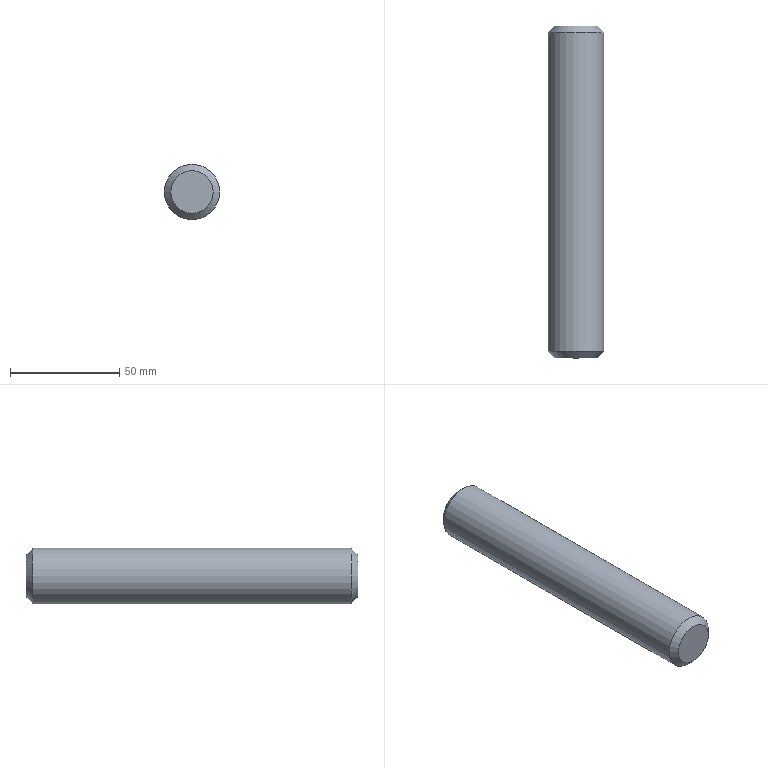Component | NX | PIN_152 | 1 solid | 5 faces | volume 76358 mm3 | plane 2 | cone 2 | cylinder 1 | commonest cylinder face diameters 25.4 x1